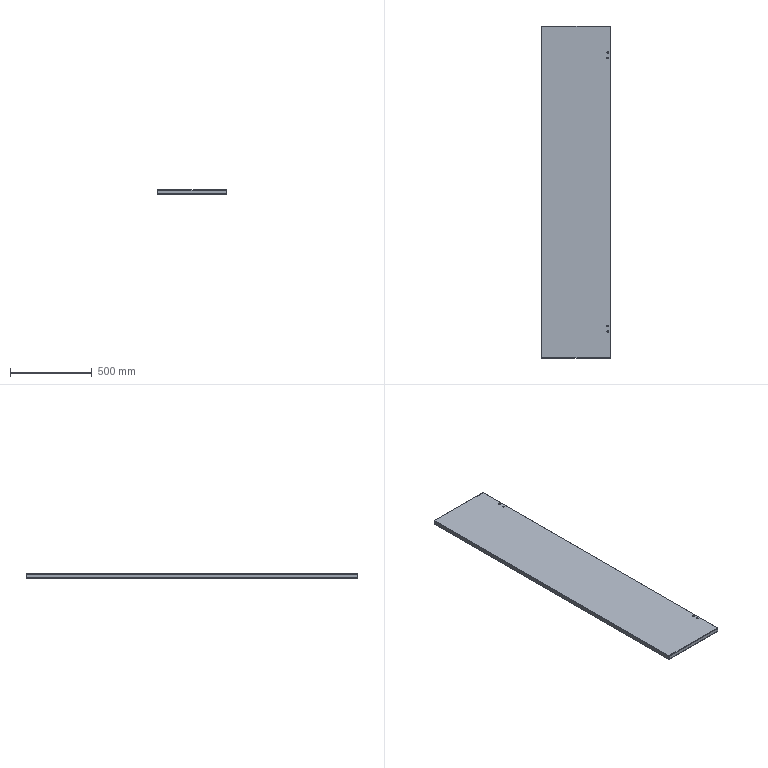Component | SolidWorks | 37ResistorRightFrontDoor-1 | 1 solid | 78 faces | volume 2009804 mm3 | plane 38 | cylinder 24 | spline 16 | commonest cylinder face diameters 10 x8 2 x8 6 x8